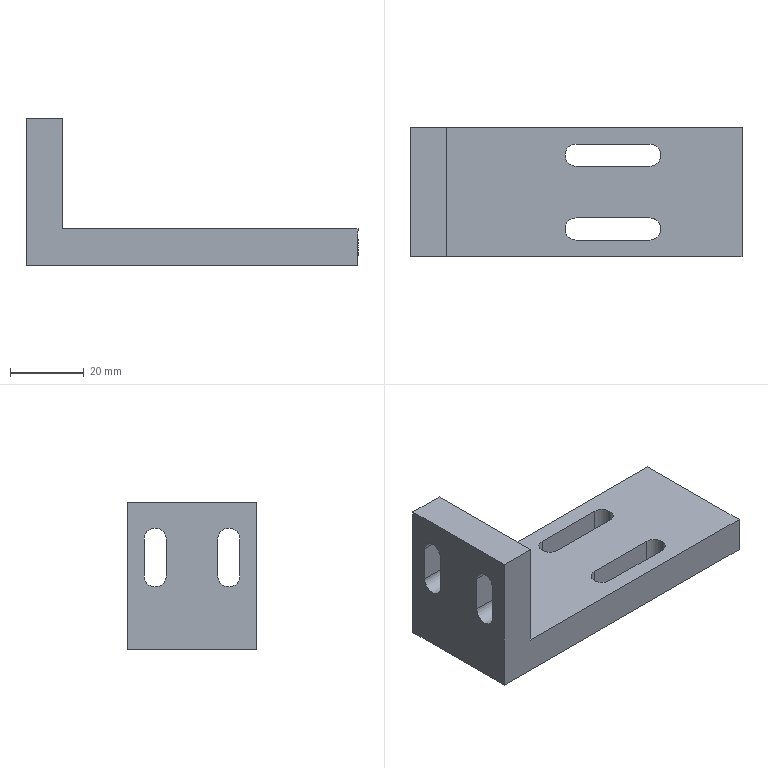Component | SolidWorks | ElectricalBoxAssembly2-1_AngleSensorComponentAssembly3-1_AdjustmentSeat-1 | 1 solid | 34 faces | box 90 x 35 x 40 mm | volume 36914 mm3 | plane 16 | cylinder 14 | cone 4 | commonest cylinder face diameters 6 x10 4.2 x4
build123d program:
from build123d import *

# Parameters (mm, degrees)
BOSS_EXTRUDE1_DEPTH   = 17.5
CUT_EXTRUDE1_DEPTH    = 92.139
CUT_EXTRUDE2_DEPTH    = 97.469
M5_TAPPED_HOLE1_D     = 4.2
M5_TAPPED_HOLE1_DEPTH = 12.4
M5_TAPPED_HOLE1_TIP   = 1.262


with BuildPart() as part:
    # Sketch1 → Boss-Extrude1 (new, symmetric)
    with BuildSketch(Plane.XY):
        Polygon((0, 0), (0, 90), (10, 90), (10, 10), (40, 10), (40, 0), align=None)
    extrude(amount=BOSS_EXTRUDE1_DEPTH, both=True)

    # Sketch2 → Cut-Extrude1 (cut, through all)
    with BuildSketch(Plane(origin=(0, 10, 0), x_dir=(1, 0, 0), z_dir=(0, 1, 0))):
        with BuildLine():
            Line((20, 13), (30, 13))
            ThreePointArc((30, 13), (33, 10), (30, 7))
            Line((30, 7), (20, 7))
            ThreePointArc((20, 7), (17, 10), (20, 13))
        make_face()
        with BuildLine():
            Line((20, -7), (30, -7))
            ThreePointArc((30, -7), (33, -10), (30, -13))
            Line((30, -13), (20, -13))
            ThreePointArc((20, -13), (17, -10), (20, -7))
        make_face()
    extrude(amount=-CUT_EXTRUDE1_DEPTH, mode=Mode.SUBTRACT)

    # Sketch3 → Cut-Extrude2 (cut, through all)
    with BuildSketch(Plane(origin=(10, 0, 0), x_dir=(0, 0, -1), z_dir=(1, 0, 0))):
        with BuildLine():
            Line((-7, 65), (-7, 45))
            ThreePointArc((-7, 45), (-10, 42), (-13, 45))
            Line((-13, 45), (-13, 65))
            ThreePointArc((-13, 65), (-10, 68), (-7, 65))
        make_face()
        with BuildLine():
            Line((13, 65), (13, 45))
            ThreePointArc((13, 45), (10, 42), (7, 45))
            Line((7, 45), (7, 65))
            ThreePointArc((7, 65), (10, 68), (13, 65))
        make_face()
    extrude(amount=-CUT_EXTRUDE2_DEPTH, mode=Mode.SUBTRACT)

    # M5 Tapped Hole1
    with Locations(Plane(origin=(0, 90, 0), x_dir=(1, 0, 0), z_dir=(0, 1, 0))):
        with Locations((5, 10), (5, -10)):
            Hole(M5_TAPPED_HOLE1_D / 2, depth=M5_TAPPED_HOLE1_DEPTH)
            with Locations((0, 0, -(M5_TAPPED_HOLE1_DEPTH + M5_TAPPED_HOLE1_TIP / 2))):  # 118° drill point
                Cone(0, M5_TAPPED_HOLE1_D / 2, M5_TAPPED_HOLE1_TIP, mode=Mode.SUBTRACT)


solid = part.part

# Placed as in the assembly
solid = solid.moved(Location((769.115, 214.666, 1766.399), (-90, 0, -90)))
STEP:
#1=COLOUR_RGB('',0.7922,0.8196,0.9333);
#2=FILL_AREA_STYLE_COLOUR('',#1);
#3=FILL_AREA_STYLE('',(#2));
#4=SURFACE_STYLE_FILL_AREA(#3);
#5=SURFACE_SIDE_STYLE('',(#4));
#6=SURFACE_STYLE_USAGE(.BOTH.,#5);
#7=PRESENTATION_STYLE_ASSIGNMENT((#6));
#8=CARTESIAN_POINT('',(33.335,7.975,69.74));
#9=VERTEX_POINT('',#8);
#10=CARTESIAN_POINT('',(33.335,8.14,69.74));
#11=VERTEX_POINT('',#10);
#12=CARTESIAN_POINT('',(33.335,8.058,69.74));
#13=DIRECTION('',(1.,0.,-0.));
#14=DIRECTION('',(0.,1.,0.));
#15=AXIS2_PLACEMENT_3D('',#12,#13,#14);
#16=CIRCLE('',#15,0.08268);
#17=EDGE_CURVE('',#9,#11,#16,.T.);
#18=ORIENTED_EDGE('',*,*,#17,.F.);
#19=CARTESIAN_POINT('',(33.823,7.975,69.74));
#20=VERTEX_POINT('',#19);
#21=CARTESIAN_POINT('',(33.823,7.975,69.74));
#22=DIRECTION('',(1.,0.,-0.));
#23=VECTOR('',#22,39.37);
#24=LINE('',#21,#23);
#25=EDGE_CURVE('',#9,#20,#24,.T.);
#26=ORIENTED_EDGE('',*,*,#25,.T.);
#27=CARTESIAN_POINT('',(33.823,8.14,69.74));
#28=VERTEX_POINT('',#27);
#29=CARTESIAN_POINT('',(33.823,8.058,69.74));
#30=DIRECTION('',(1.,0.,-0.));
#31=DIRECTION('',(0.,1.,0.));
#32=AXIS2_PLACEMENT_3D('',#29,#30,#31);
#33=CIRCLE('',#32,0.08268);
#34=EDGE_CURVE('',#20,#28,#33,.T.);
#35=ORIENTED_EDGE('',*,*,#34,.T.);
#36=CARTESIAN_POINT('',(33.823,8.14,69.74));
#37=DIRECTION('',(1.,0.,-0.));
#38=VECTOR('',#37,39.37);
#39=LINE('',#36,#38);
#40=EDGE_CURVE('',#11,#28,#39,.T.);
#41=ORIENTED_EDGE('',*,*,#40,.F.);
#42=EDGE_LOOP('',(#18,#26,#35,#41));
#43=FACE_OUTER_BOUND('',#42,.T.);
#44=CARTESIAN_POINT('',(33.823,8.058,69.74));
#45=DIRECTION('',(1.,0.,-0.));
#46=DIRECTION('',(0.,1.,0.));
#47=AXIS2_PLACEMENT_3D('',#44,#45,#46);
#48=CYLINDRICAL_SURFACE('',#47,0.08268);
#49=ADVANCED_FACE('',(#43),#48,.F.);
#50=CARTESIAN_POINT('',(33.286,8.058,69.74));
#51=VERTEX_POINT('',#50);
#52=CARTESIAN_POINT('',(33.335,8.14,69.74));
#53=DIRECTION('',(0.515,0.8572,-0.));
#54=VECTOR('',#53,39.37);
#55=LINE('',#52,#54);
#56=EDGE_CURVE('',#51,#11,#55,.T.);
#57=ORIENTED_EDGE('',*,*,#56,.F.);
#58=CARTESIAN_POINT('',(33.335,7.975,69.74));
#59=DIRECTION('',(0.515,-0.8572,-0.));
#60=VECTOR('',#59,39.37);
#61=LINE('',#58,#60);
#62=EDGE_CURVE('',#51,#9,#61,.T.);
#63=ORIENTED_EDGE('',*,*,#62,.T.);
#64=ORIENTED_EDGE('',*,*,#17,.T.);
#65=EDGE_LOOP('',(#57,#63,#64));
#66=FACE_OUTER_BOUND('',#65,.T.);
#67=CARTESIAN_POINT('',(33.335,8.058,69.74));
#68=DIRECTION('',(1.,0.,-0.));
#69=DIRECTION('',(0.,1.,0.));
#70=AXIS2_PLACEMENT_3D('',#67,#68,#69);
#71=CONICAL_SURFACE('',#70,0.08268,1.03);
#72=ADVANCED_FACE('',(#66),#71,.F.);
#73=CARTESIAN_POINT('',(33.335,8.762,69.74));
#74=VERTEX_POINT('',#73);
#75=CARTESIAN_POINT('',(33.335,8.928,69.74));
#76=VERTEX_POINT('',#75);
#77=CARTESIAN_POINT('',(33.335,8.845,69.74));
#78=DIRECTION('',(1.,0.,-0.));
#79=DIRECTION('',(0.,1.,0.));
#80=AXIS2_PLACEMENT_3D('',#77,#78,#79);
#81=CIRCLE('',#80,0.08268);
#82=EDGE_CURVE('',#74,#76,#81,.T.);
#83=ORIENTED_EDGE('',*,*,#82,.F.);
#84=CARTESIAN_POINT('',(33.823,8.762,69.74));
#85=VERTEX_POINT('',#84);
#86=CARTESIAN_POINT('',(33.823,8.762,69.74));
#87=DIRECTION('',(1.,0.,-0.));
#88=VECTOR('',#87,39.37);
#89=LINE('',#86,#88);
#90=EDGE_CURVE('',#74,#85,#89,.T.);
#91=ORIENTED_EDGE('',*,*,#90,.T.);
#92=CARTESIAN_POINT('',(33.823,8.928,69.74));
#93=VERTEX_POINT('',#92);
#94=CARTESIAN_POINT('',(33.823,8.845,69.74));
#95=DIRECTION('',(1.,0.,-0.));
#96=DIRECTION('',(0.,1.,0.));
#97=AXIS2_PLACEMENT_3D('',#94,#95,#96);
#98=CIRCLE('',#97,0.08268);
#99=EDGE_CURVE('',#85,#93,#98,.T.);
#100=ORIENTED_EDGE('',*,*,#99,.T.);
#101=CARTESIAN_POINT('',(33.823,8.928,69.74));
#102=DIRECTION('',(1.,0.,-0.));
#103=VECTOR('',#102,39.37);
#104=LINE('',#101,#103);
#105=EDGE_CURVE('',#76,#93,#104,.T.);
#106=ORIENTED_EDGE('',*,*,#105,.F.);
#107=EDGE_LOOP('',(#83,#91,#100,#106));
#108=FACE_OUTER_BOUND('',#107,.T.);
#109=CARTESIAN_POINT('',(33.823,8.845,69.74));
#110=DIRECTION('',(1.,0.,-0.));
#111=DIRECTION('',(0.,1.,0.));
#112=AXIS2_PLACEMENT_3D('',#109,#110,#111);
#113=CYLINDRICAL_SURFACE('',#112,0.08268);
#114=ADVANCED_FACE('',(#108),#113,.F.);
#115=CARTESIAN_POINT('',(33.286,8.845,69.74));
#116=VERTEX_POINT('',#115);
#117=CARTESIAN_POINT('',(33.335,8.928,69.74));
#118=DIRECTION('',(0.515,0.8572,-0.));
#119=VECTOR('',#118,39.37);
#120=LINE('',#117,#119);
#121=EDGE_CURVE('',#116,#76,#120,.T.);
#122=ORIENTED_EDGE('',*,*,#121,.F.);
#123=CARTESIAN_POINT('',(33.335,8.762,69.74));
#124=DIRECTION('',(0.515,-0.8572,-0.));
#125=VECTOR('',#124,39.37);
#126=LINE('',#123,#125);
#127=EDGE_CURVE('',#116,#74,#126,.T.);
#128=ORIENTED_EDGE('',*,*,#127,.T.);
#129=ORIENTED_EDGE('',*,*,#82,.T.);
#130=EDGE_LOOP('',(#122,#128,#129));
#131=FACE_OUTER_BOUND('',#130,.T.);
#132=CARTESIAN_POINT('',(33.335,8.845,69.74));
#133=DIRECTION('',(1.,0.,-0.));
#134=DIRECTION('',(0.,1.,0.));
#135=AXIS2_PLACEMENT_3D('',#132,#133,#134);
#136=CONICAL_SURFACE('',#135,0.08268,1.03);
#137=ADVANCED_FACE('',(#131),#136,.F.);
#138=CARTESIAN_POINT('',(32.957,8.058,69.543));
#139=VERTEX_POINT('',#138);
#140=CARTESIAN_POINT('',(32.839,8.176,69.543));
#141=VERTEX_POINT('',#140);
#142=CARTESIAN_POINT('',(32.839,8.058,69.543));
#143=DIRECTION('',(0.,0.,1.));
#144=DIRECTION('',(1.,0.,0.));
#145=AXIS2_PLACEMENT_3D('',#142,#143,#144);
#146=CIRCLE('',#145,0.1181);
#147=EDGE_CURVE('',#139,#141,#146,.T.);
#148=ORIENTED_EDGE('',*,*,#147,.F.);
#149=CARTESIAN_POINT('',(32.957,8.058,69.937));
#150=VERTEX_POINT('',#149);
#151=CARTESIAN_POINT('',(32.957,8.058,69.543));
#152=DIRECTION('',(0.,0.,1.));
#153=VECTOR('',#152,39.37);
#154=LINE('',#151,#153);
#155=EDGE_CURVE('',#139,#150,#154,.T.);
#156=ORIENTED_EDGE('',*,*,#155,.T.);
#157=CARTESIAN_POINT('',(32.839,8.176,69.937));
#158=VERTEX_POINT('',#157);
#159=CARTESIAN_POINT('',(32.839,8.058,69.937));
#160=DIRECTION('',(0.,0.,1.));
#161=DIRECTION('',(1.,0.,0.));
#162=AXIS2_PLACEMENT_3D('',#159,#160,#161);
#163=CIRCLE('',#162,0.1181);
#164=EDGE_CURVE('',#150,#158,#163,.T.);
#165=ORIENTED_EDGE('',*,*,#164,.T.);
#166=CARTESIAN_POINT('',(32.839,8.176,69.543));
#167=DIRECTION('',(0.,0.,1.));
#168=VECTOR('',#167,39.37);
#169=LINE('',#166,#168);
#170=EDGE_CURVE('',#141,#158,#169,.T.);
#171=ORIENTED_EDGE('',*,*,#170,.F.);
#172=EDGE_LOOP('',(#148,#156,#165,#171));
#173=FACE_OUTER_BOUND('',#172,.T.);
#174=CARTESIAN_POINT('',(32.839,8.058,69.543));
#175=DIRECTION('',(0.,0.,1.));
#176=DIRECTION('',(1.,0.,0.));
#177=AXIS2_PLACEMENT_3D('',#174,#175,#176);
#178=CYLINDRICAL_SURFACE('',#177,0.1181);
#179=ADVANCED_FACE('',(#173),#178,.F.);
#180=CARTESIAN_POINT('',(32.957,8.845,69.543));
#181=VERTEX_POINT('',#180);
#182=CARTESIAN_POINT('',(32.839,8.963,69.543));
#183=VERTEX_POINT('',#182);
#184=CARTESIAN_POINT('',(32.839,8.845,69.543));
#185=DIRECTION('',(0.,0.,1.));
#186=DIRECTION('',(1.,0.,0.));
#187=AXIS2_PLACEMENT_3D('',#184,#185,#186);
#188=CIRCLE('',#187,0.1181);
#189=EDGE_CURVE('',#181,#183,#188,.T.);
#190=ORIENTED_EDGE('',*,*,#189,.F.);
#191=CARTESIAN_POINT('',(32.957,8.845,69.937));
#192=VERTEX_POINT('',#191);
#193=CARTESIAN_POINT('',(32.957,8.845,69.543));
#194=DIRECTION('',(0.,0.,1.));
#195=VECTOR('',#194,39.37);
#196=LINE('',#193,#195);
#197=EDGE_CURVE('',#181,#192,#196,.T.);
#198=ORIENTED_EDGE('',*,*,#197,.T.);
#199=CARTESIAN_POINT('',(32.839,8.963,69.937));
#200=VERTEX_POINT('',#199);
#201=CARTESIAN_POINT('',(32.839,8.845,69.937));
#202=DIRECTION('',(0.,0.,1.));
#203=DIRECTION('',(1.,0.,0.));
#204=AXIS2_PLACEMENT_3D('',#201,#202,#203);
#205=CIRCLE('',#204,0.1181);
#206=EDGE_CURVE('',#192,#200,#205,.T.);
#207=ORIENTED_EDGE('',*,*,#206,.T.);
#208=CARTESIAN_POINT('',(32.839,8.963,69.543));
#209=DIRECTION('',(0.,0.,1.));
#210=VECTOR('',#209,39.37);
#211=LINE('',#208,#210);
#212=EDGE_CURVE('',#183,#200,#211,.T.);
#213=ORIENTED_EDGE('',*,*,#212,.F.);
#214=EDGE_LOOP('',(#190,#198,#207,#213));
#215=FACE_OUTER_BOUND('',#214,.T.);
#216=CARTESIAN_POINT('',(32.839,8.845,69.543));
#217=DIRECTION('',(0.,0.,1.));
#218=DIRECTION('',(1.,0.,0.));
#219=AXIS2_PLACEMENT_3D('',#216,#217,#218);
#220=CYLINDRICAL_SURFACE('',#219,0.1181);
#221=ADVANCED_FACE('',(#215),#220,.F.);
#222=CARTESIAN_POINT('',(30.28,8.727,70.724));
#223=VERTEX_POINT('',#222);
#224=CARTESIAN_POINT('',(30.28,8.727,70.331));
#225=VERTEX_POINT('',#224);
#226=CARTESIAN_POINT('',(30.28,8.727,70.331));
#227=DIRECTION('',(-0.,-0.,-1.));
#228=VECTOR('',#227,39.37);
#229=LINE('',#226,#228);
#230=EDGE_CURVE('',#223,#225,#229,.T.);
#231=ORIENTED_EDGE('',*,*,#230,.T.);
#232=CARTESIAN_POINT('',(30.28,8.963,70.331));
#233=VERTEX_POINT('',#232);
#234=CARTESIAN_POINT('',(30.28,8.845,70.331));
#235=DIRECTION('',(1.,0.,-0.));
#236=DIRECTION('',(0.,1.,0.));
#237=AXIS2_PLACEMENT_3D('',#234,#235,#236);
#238=CIRCLE('',#237,0.1181);
#239=EDGE_CURVE('',#225,#233,#238,.T.);
#240=ORIENTED_EDGE('',*,*,#239,.T.);
#241=CARTESIAN_POINT('',(30.28,8.963,70.724));
#242=VERTEX_POINT('',#241);
#243=CARTESIAN_POINT('',(30.28,8.963,70.331));
#244=DIRECTION('',(0.,0.,1.));
#245=VECTOR('',#244,39.37);
#246=LINE('',#243,#245);
#247=EDGE_CURVE('',#233,#242,#246,.T.);
#248=ORIENTED_EDGE('',*,*,#247,.T.);
#249=CARTESIAN_POINT('',(30.28,8.845,70.724));
#250=DIRECTION('',(1.,0.,-0.));
#251=DIRECTION('',(0.,1.,0.));
#252=AXIS2_PLACEMENT_3D('',#249,#250,#251);
#253=CIRCLE('',#252,0.1181);
#254=EDGE_CURVE('',#242,#223,#253,.T.);
#255=ORIENTED_EDGE('',*,*,#254,.T.);
#256=EDGE_LOOP('',(#231,#240,#248,#255));
#257=FACE_BOUND('',#256,.T.);
#258=CARTESIAN_POINT('',(30.28,7.94,70.724));
#259=VERTEX_POINT('',#258);
#260=CARTESIAN_POINT('',(30.28,7.94,70.331));
#261=VERTEX_POINT('',#260);
#262=CARTESIAN_POINT('',(30.28,7.94,70.331));
#263=DIRECTION('',(-0.,-0.,-1.));
#264=VECTOR('',#263,39.37);
#265=LINE('',#262,#264);
#266=EDGE_CURVE('',#259,#261,#265,.T.);
#267=ORIENTED_EDGE('',*,*,#266,.T.);
#268=CARTESIAN_POINT('',(30.28,8.176,70.331));
#269=VERTEX_POINT('',#268);
#270=CARTESIAN_POINT('',(30.28,8.058,70.331));
#271=DIRECTION('',(1.,0.,-0.));
#272=DIRECTION('',(0.,1.,0.));
#273=AXIS2_PLACEMENT_3D('',#270,#271,#272);
#274=CIRCLE('',#273,0.1181);
#275=EDGE_CURVE('',#261,#269,#274,.T.);
#276=ORIENTED_EDGE('',*,*,#275,.T.);
#277=CARTESIAN_POINT('',(30.28,8.176,70.724));
#278=VERTEX_POINT('',#277);
#279=CARTESIAN_POINT('',(30.28,8.176,70.331));
#280=DIRECTION('',(0.,0.,1.));
#281=VECTOR('',#280,39.37);
#282=LINE('',#279,#281);
#283=EDGE_CURVE('',#269,#278,#282,.T.);
#284=ORIENTED_EDGE('',*,*,#283,.T.);
#285=CARTESIAN_POINT('',(30.28,8.058,70.724));
#286=DIRECTION('',(1.,0.,-0.));
#287=DIRECTION('',(0.,1.,0.));
#288=AXIS2_PLACEMENT_3D('',#285,#286,#287);
#289=CIRCLE('',#288,0.1181);
#290=EDGE_CURVE('',#278,#259,#289,.T.);
#291=ORIENTED_EDGE('',*,*,#290,.T.);
#292=EDGE_LOOP('',(#267,#276,#284,#291));
#293=FACE_BOUND('',#292,.T.);
#294=CARTESIAN_POINT('',(30.28,7.762,69.543));
#295=VERTEX_POINT('',#294);
#296=CARTESIAN_POINT('',(30.28,7.762,71.118));
#297=VERTEX_POINT('',#296);
#298=CARTESIAN_POINT('',(30.28,7.762,71.118));
#299=DIRECTION('',(0.,0.,1.));
#300=VECTOR('',#299,39.37);
#301=LINE('',#298,#300);
#302=EDGE_CURVE('',#295,#297,#301,.T.);
#303=ORIENTED_EDGE('',*,*,#302,.T.);
#304=CARTESIAN_POINT('',(30.28,9.14,71.118));
#305=VERTEX_POINT('',#304);
#306=CARTESIAN_POINT('',(30.28,9.14,71.118));
#307=DIRECTION('',(0.,-1.,0.));
#308=VECTOR('',#307,39.37);
#309=LINE('',#306,#308);
#310=EDGE_CURVE('',#305,#297,#309,.T.);
#311=ORIENTED_EDGE('',*,*,#310,.F.);
#312=CARTESIAN_POINT('',(30.28,9.14,69.543));
#313=VERTEX_POINT('',#312);
#314=CARTESIAN_POINT('',(30.28,9.14,71.118));
#315=DIRECTION('',(0.,0.,1.));
#316=VECTOR('',#315,39.37);
#317=LINE('',#314,#316);
#318=EDGE_CURVE('',#313,#305,#317,.T.);
#319=ORIENTED_EDGE('',*,*,#318,.F.);
#320=CARTESIAN_POINT('',(30.28,9.14,69.543));
#321=DIRECTION('',(0.,-1.,0.));
#322=VECTOR('',#321,39.37);
#323=LINE('',#320,#322);
#324=EDGE_CURVE('',#313,#295,#323,.T.);
#325=ORIENTED_EDGE('',*,*,#324,.T.);
#326=EDGE_LOOP('',(#303,#311,#319,#325));
#327=FACE_OUTER_BOUND('',#326,.T.);
#328=CARTESIAN_POINT('',(30.28,9.14,71.118));
#329=DIRECTION('',(1.,0.,-0.));
#330=DIRECTION('',(-0.,-0.,-1.));
#331=AXIS2_PLACEMENT_3D('',#328,#329,#330);
#332=PLANE('',#331);
#333=ADVANCED_FACE('',(#257,#293,#327),#332,.F.);
#334=CARTESIAN_POINT('',(30.674,7.762,71.118));
#335=VERTEX_POINT('',#334);
#336=CARTESIAN_POINT('',(30.674,7.762,71.118));
#337=DIRECTION('',(1.,0.,-0.));
#338=VECTOR('',#337,39.37);
#339=LINE('',#336,#338);
#340=EDGE_CURVE('',#297,#335,#339,.T.);
#341=ORIENTED_EDGE('',*,*,#340,.T.);
#342=CARTESIAN_POINT('',(30.674,9.14,71.118));
#343=VERTEX_POINT('',#342);
#344=CARTESIAN_POINT('',(30.674,9.14,71.118));
#345=DIRECTION('',(0.,-1.,0.));
#346=VECTOR('',#345,39.37);
#347=LINE('',#344,#346);
#348=EDGE_CURVE('',#343,#335,#347,.T.);
#349=ORIENTED_EDGE('',*,*,#348,.F.);
#350=CARTESIAN_POINT('',(30.674,9.14,71.118));
#351=DIRECTION('',(1.,0.,-0.));
#352=VECTOR('',#351,39.37);
#353=LINE('',#350,#352);
#354=EDGE_CURVE('',#305,#343,#353,.T.);
#355=ORIENTED_EDGE('',*,*,#354,.F.);
#356=ORIENTED_EDGE('',*,*,#310,.T.);
#357=EDGE_LOOP('',(#341,#349,#355,#356));
#358=FACE_OUTER_BOUND('',#357,.T.);
#359=CARTESIAN_POINT('',(30.674,9.14,71.118));
#360=DIRECTION('',(-0.,-0.,-1.));
#361=DIRECTION('',(-0.,1.,-0.));
#362=AXIS2_PLACEMENT_3D('',#359,#360,#361);
#363=PLANE('',#362);
#364=ADVANCED_FACE('',(#358),#363,.F.);
#365=CARTESIAN_POINT('',(30.674,8.963,70.331));
#366=VERTEX_POINT('',#365);
#367=CARTESIAN_POINT('',(30.674,8.963,70.724));
#368=VERTEX_POINT('',#367);
#369=CARTESIAN_POINT('',(30.674,8.963,70.331));
#370=DIRECTION('',(0.,0.,1.));
#371=VECTOR('',#370,39.37);
#372=LINE('',#369,#371);
#373=EDGE_CURVE('',#366,#368,#372,.T.);
#374=ORIENTED_EDGE('',*,*,#373,.F.);
#375=CARTESIAN_POINT('',(30.674,8.727,70.331));
#376=VERTEX_POINT('',#375);
#377=CARTESIAN_POINT('',(30.674,8.845,70.331));
#378=DIRECTION('',(1.,0.,-0.));
#379=DIRECTION('',(0.,1.,0.));
#380=AXIS2_PLACEMENT_3D('',#377,#378,#379);
#381=CIRCLE('',#380,0.1181);
#382=EDGE_CURVE('',#376,#366,#381,.T.);
#383=ORIENTED_EDGE('',*,*,#382,.F.);
#384=CARTESIAN_POINT('',(30.674,8.727,70.724));
#385=VERTEX_POINT('',#384);
#386=CARTESIAN_POINT('',(30.674,8.727,70.331));
#387=DIRECTION('',(-0.,-0.,-1.));
#388=VECTOR('',#387,39.37);
#389=LINE('',#386,#388);
#390=EDGE_CURVE('',#385,#376,#389,.T.);
#391=ORIENTED_EDGE('',*,*,#390,.F.);
#392=CARTESIAN_POINT('',(30.674,8.845,70.724));
#393=DIRECTION('',(1.,0.,-0.));
#394=DIRECTION('',(0.,1.,0.));
#395=AXIS2_PLACEMENT_3D('',#392,#393,#394);
#396=CIRCLE('',#395,0.1181);
#397=EDGE_CURVE('',#368,#385,#396,.T.);
#398=ORIENTED_EDGE('',*,*,#397,.F.);
#399=EDGE_LOOP('',(#374,#383,#391,#398));
#400=FACE_BOUND('',#399,.T.);
#401=CARTESIAN_POINT('',(30.674,8.176,70.331));
#402=VERTEX_POINT('',#401);
#403=CARTESIAN_POINT('',(30.674,8.176,70.724));
#404=VERTEX_POINT('',#403);
#405=CARTESIAN_POINT('',(30.674,8.176,70.331));
#406=DIRECTION('',(0.,0.,1.));
#407=VECTOR('',#406,39.37);
#408=LINE('',#405,#407);
#409=EDGE_CURVE('',#402,#404,#408,.T.);
#410=ORIENTED_EDGE('',*,*,#409,.F.);
#411=CARTESIAN_POINT('',(30.674,7.94,70.331));
#412=VERTEX_POINT('',#411);
#413=CARTESIAN_POINT('',(30.674,8.058,70.331));
#414=DIRECTION('',(1.,0.,-0.));
#415=DIRECTION('',(0.,1.,0.));
#416=AXIS2_PLACEMENT_3D('',#413,#414,#415);
#417=CIRCLE('',#416,0.1181);
#418=EDGE_CURVE('',#412,#402,#417,.T.);
#419=ORIENTED_EDGE('',*,*,#418,.F.);
#420=CARTESIAN_POINT('',(30.674,7.94,70.724));
#421=VERTEX_POINT('',#420);
#422=CARTESIAN_POINT('',(30.674,7.94,70.331));
#423=DIRECTION('',(-0.,-0.,-1.));
#424=VECTOR('',#423,39.37);
#425=LINE('',#422,#424);
#426=EDGE_CURVE('',#421,#412,#425,.T.);
#427=ORIENTED_EDGE('',*,*,#426,.F.);
#428=CARTESIAN_POINT('',(30.674,8.058,70.724));
#429=DIRECTION('',(1.,0.,-0.));
#430=DIRECTION('',(0.,1.,0.));
#431=AXIS2_PLACEMENT_3D('',#428,#429,#430);
#432=CIRCLE('',#431,0.1181);
#433=EDGE_CURVE('',#404,#421,#432,.T.);
#434=ORIENTED_EDGE('',*,*,#433,.F.);
#435=EDGE_LOOP('',(#410,#419,#427,#434));
#436=FACE_BOUND('',#435,.T.);
#437=CARTESIAN_POINT('',(30.674,7.762,69.937));
#438=VERTEX_POINT('',#437);
#439=CARTESIAN_POINT('',(30.674,7.762,69.937));
#440=DIRECTION('',(-0.,-0.,-1.));
#441=VECTOR('',#440,39.37);
#442=LINE('',#439,#441);
#443=EDGE_CURVE('',#335,#438,#442,.T.);
#444=ORIENTED_EDGE('',*,*,#443,.T.);
#445=CARTESIAN_POINT('',(30.674,9.14,69.937));
#446=VERTEX_POINT('',#445);
#447=CARTESIAN_POINT('',(30.674,9.14,69.937));
#448=DIRECTION('',(0.,-1.,0.));
#449=VECTOR('',#448,39.37);
#450=LINE('',#447,#449);
#451=EDGE_CURVE('',#446,#438,#450,.T.);
#452=ORIENTED_EDGE('',*,*,#451,.F.);
#453=CARTESIAN_POINT('',(30.674,9.14,69.937));
#454=DIRECTION('',(-0.,-0.,-1.));
#455=VECTOR('',#454,39.37);
#456=LINE('',#453,#455);
#457=EDGE_CURVE('',#343,#446,#456,.T.);
#458=ORIENTED_EDGE('',*,*,#457,.F.);
#459=ORIENTED_EDGE('',*,*,#348,.T.);
#460=EDGE_LOOP('',(#444,#452,#458,#459));
#461=FACE_OUTER_BOUND('',#460,.T.);
#462=CARTESIAN_POINT('',(30.674,9.14,69.937));
#463=DIRECTION('',(-1.,0.,0.));
#464=DIRECTION('',(0.,-1.,0.));
#465=AXIS2_PLACEMENT_3D('',#462,#463,#464);
#466=PLANE('',#465);
#467=ADVANCED_FACE('',(#400,#436,#461),#466,.F.);
#468=CARTESIAN_POINT('',(32.052,8.176,69.937));
#469=VERTEX_POINT('',#468);
#470=CARTESIAN_POINT('',(32.839,8.176,69.937));
#471=DIRECTION('',(-1.,-0.,0.));
#472=VECTOR('',#471,39.37);
#473=LINE('',#470,#472);
#474=EDGE_CURVE('',#158,#469,#473,.T.);
#475=ORIENTED_EDGE('',*,*,#474,.F.);
#476=ORIENTED_EDGE('',*,*,#164,.F.);
#477=CARTESIAN_POINT('',(32.839,7.94,69.937));
#478=VERTEX_POINT('',#477);
#479=CARTESIAN_POINT('',(32.839,8.058,69.937));
#480=DIRECTION('',(0.,0.,1.));
#481=DIRECTION('',(1.,0.,0.));
#482=AXIS2_PLACEMENT_3D('',#479,#480,#481);
#483=CIRCLE('',#482,0.1181);
#484=EDGE_CURVE('',#478,#150,#483,.T.);
#485=ORIENTED_EDGE('',*,*,#484,.F.);
#486=CARTESIAN_POINT('',(32.052,7.94,69.937));
#487=VERTEX_POINT('',#486);
#488=CARTESIAN_POINT('',(32.839,7.94,69.937));
#489=DIRECTION('',(1.,0.,-0.));
#490=VECTOR('',#489,39.37);
#491=LINE('',#488,#490);
#492=EDGE_CURVE('',#487,#478,#491,.T.);
#493=ORIENTED_EDGE('',*,*,#492,.F.);
#494=CARTESIAN_POINT('',(32.052,8.058,69.937));
#495=DIRECTION('',(0.,0.,1.));
#496=DIRECTION('',(1.,0.,0.));
#497=AXIS2_PLACEMENT_3D('',#494,#495,#496);
#498=CIRCLE('',#497,0.1181);
#499=EDGE_CURVE('',#469,#487,#498,.T.);
#500=ORIENTED_EDGE('',*,*,#499,.F.);
#501=EDGE_LOOP('',(#475,#476,#485,#493,#500));
#502=FACE_BOUND('',#501,.T.);
#503=CARTESIAN_POINT('',(32.052,8.963,69.937));
#504=VERTEX_POINT('',#503);
#505=CARTESIAN_POINT('',(32.839,8.963,69.937));
#506=DIRECTION('',(-1.,-0.,0.));
#507=VECTOR('',#506,39.37);
#508=LINE('',#505,#507);
#509=EDGE_CURVE('',#200,#504,#508,.T.);
#510=ORIENTED_EDGE('',*,*,#509,.F.);
#511=ORIENTED_EDGE('',*,*,#206,.F.);
#512=CARTESIAN_POINT('',(32.839,8.727,69.937));
#513=VERTEX_POINT('',#512);
#514=CARTESIAN_POINT('',(32.839,8.845,69.937));
#515=DIRECTION('',(0.,0.,1.));
#516=DIRECTION('',(1.,0.,0.));
#517=AXIS2_PLACEMENT_3D('',#514,#515,#516);
#518=CIRCLE('',#517,0.1181);
#519=EDGE_CURVE('',#513,#192,#518,.T.);
#520=ORIENTED_EDGE('',*,*,#519,.F.);
#521=CARTESIAN_POINT('',(32.052,8.727,69.937));
#522=VERTEX_POINT('',#521);
#523=CARTESIAN_POINT('',(32.839,8.727,69.937));
#524=DIRECTION('',(1.,0.,-0.));
#525=VECTOR('',#524,39.37);
#526=LINE('',#523,#525);
#527=EDGE_CURVE('',#522,#513,#526,.T.);
#528=ORIENTED_EDGE('',*,*,#527,.F.);
#529=CARTESIAN_POINT('',(32.052,8.845,69.937));
#530=DIRECTION('',(0.,0.,1.));
#531=DIRECTION('',(1.,0.,0.));
#532=AXIS2_PLACEMENT_3D('',#529,#530,#531);
#533=CIRCLE('',#532,0.1181);
#534=EDGE_CURVE('',#504,#522,#533,.T.);
#535=ORIENTED_EDGE('',*,*,#534,.F.);
#536=EDGE_LOOP('',(#510,#511,#520,#528,#535));
#537=FACE_BOUND('',#536,.T.);
#538=CARTESIAN_POINT('',(33.823,7.762,69.937));
#539=VERTEX_POINT('',#538);
#540=CARTESIAN_POINT('',(33.823,7.762,69.937));
#541=DIRECTION('',(1.,0.,-0.));
#542=VECTOR('',#541,39.37);
#543=LINE('',#540,#542);
#544=EDGE_CURVE('',#438,#539,#543,.T.);
#545=ORIENTED_EDGE('',*,*,#544,.T.);
#546=CARTESIAN_POINT('',(33.823,9.14,69.937));
#547=VERTEX_POINT('',#546);
#548=CARTESIAN_POINT('',(33.823,9.14,69.937));
#549=DIRECTION('',(0.,-1.,0.));
#550=VECTOR('',#549,39.37);
#551=LINE('',#548,#550);
#552=EDGE_CURVE('',#547,#539,#551,.T.);
#553=ORIENTED_EDGE('',*,*,#552,.F.);
#554=CARTESIAN_POINT('',(33.823,9.14,69.937));
#555=DIRECTION('',(1.,0.,-0.));
#556=VECTOR('',#555,39.37);
#557=LINE('',#554,#556);
#558=EDGE_CURVE('',#446,#547,#557,.T.);
#559=ORIENTED_EDGE('',*,*,#558,.F.);
#560=ORIENTED_EDGE('',*,*,#451,.T.);
#561=EDGE_LOOP('',(#545,#553,#559,#560));
#562=FACE_OUTER_BOUND('',#561,.T.);
#563=CARTESIAN_POINT('',(33.823,9.14,69.937));
#564=DIRECTION('',(-0.,-0.,-1.));
#565=DIRECTION('',(-1.,-0.,0.));
#566=AXIS2_PLACEMENT_3D('',#563,#564,#565);
#567=PLANE('',#566);
#568=ADVANCED_FACE('',(#502,#537,#562),#567,.F.);
#569=CARTESIAN_POINT('',(33.823,8.058,69.74));
#570=DIRECTION('',(1.,0.,-0.));
#571=DIRECTION('',(0.,1.,0.));
#572=AXIS2_PLACEMENT_3D('',#569,#570,#571);
#573=CIRCLE('',#572,0.08268);
#574=EDGE_CURVE('',#28,#20,#573,.T.);
#575=ORIENTED_EDGE('',*,*,#574,.F.);
#576=ORIENTED_EDGE('',*,*,#34,.F.);
#577=EDGE_LOOP('',(#575,#576));
#578=FACE_BOUND('',#577,.T.);
#579=CARTESIAN_POINT('',(33.823,8.845,69.74));
#580=DIRECTION('',(1.,0.,-0.));
#581=DIRECTION('',(0.,1.,0.));
#582=AXIS2_PLACEMENT_3D('',#579,#580,#581);
#583=CIRCLE('',#582,0.08268);
#584=EDGE_CURVE('',#93,#85,#583,.T.);
#585=ORIENTED_EDGE('',*,*,#584,.F.);
#586=ORIENTED_EDGE('',*,*,#99,.F.);
#587=EDGE_LOOP('',(#585,#586));
#588=FACE_BOUND('',#587,.T.);
#589=CARTESIAN_POINT('',(33.823,7.762,69.543));
#590=VERTEX_POINT('',#589);
#591=CARTESIAN_POINT('',(33.823,7.762,69.543));
#592=DIRECTION('',(-0.,-0.,-1.));
#593=VECTOR('',#592,39.37);
#594=LINE('',#591,#593);
#595=EDGE_CURVE('',#539,#590,#594,.T.);
#596=ORIENTED_EDGE('',*,*,#595,.T.);
#597=CARTESIAN_POINT('',(33.823,9.14,69.543));
#598=VERTEX_POINT('',#597);
#599=CARTESIAN_POINT('',(33.823,9.14,69.543));
#600=DIRECTION('',(0.,-1.,0.));
#601=VECTOR('',#600,39.37);
#602=LINE('',#599,#601);
#603=EDGE_CURVE('',#598,#590,#602,.T.);
#604=ORIENTED_EDGE('',*,*,#603,.F.);
#605=CARTESIAN_POINT('',(33.823,9.14,69.543));
#606=DIRECTION('',(-0.,-0.,-1.));
#607=VECTOR('',#606,39.37);
#608=LINE('',#605,#607);
#609=EDGE_CURVE('',#547,#598,#608,.T.);
#610=ORIENTED_EDGE('',*,*,#609,.F.);
#611=ORIENTED_EDGE('',*,*,#552,.T.);
#612=EDGE_LOOP('',(#596,#604,#610,#611));
#613=FACE_OUTER_BOUND('',#612,.T.);
#614=CARTESIAN_POINT('',(33.823,9.14,69.543));
#615=DIRECTION('',(-1.,0.,0.));
#616=DIRECTION('',(0.,-1.,0.));
#617=AXIS2_PLACEMENT_3D('',#614,#615,#616);
#618=PLANE('',#617);
#619=ADVANCED_FACE('',(#578,#588,#613),#618,.F.);
#620=CARTESIAN_POINT('',(32.052,7.94,69.543));
#621=VERTEX_POINT('',#620);
#622=CARTESIAN_POINT('',(32.839,7.94,69.543));
#623=VERTEX_POINT('',#622);
#624=CARTESIAN_POINT('',(32.839,7.94,69.543));
#625=DIRECTION('',(1.,0.,-0.));
#626=VECTOR('',#625,39.37);
#627=LINE('',#624,#626);
#628=EDGE_CURVE('',#621,#623,#627,.T.);
#629=ORIENTED_EDGE('',*,*,#628,.T.);
#630=CARTESIAN_POINT('',(32.839,8.058,69.543));
#631=DIRECTION('',(0.,0.,1.));
#632=DIRECTION('',(1.,0.,0.));
#633=AXIS2_PLACEMENT_3D('',#630,#631,#632);
#634=CIRCLE('',#633,0.1181);
#635=EDGE_CURVE('',#623,#139,#634,.T.);
#636=ORIENTED_EDGE('',*,*,#635,.T.);
#637=ORIENTED_EDGE('',*,*,#147,.T.);
#638=CARTESIAN_POINT('',(32.052,8.176,69.543));
#639=VERTEX_POINT('',#638);
#640=CARTESIAN_POINT('',(32.839,8.176,69.543));
#641=DIRECTION('',(-1.,-0.,0.));
#642=VECTOR('',#641,39.37);
#643=LINE('',#640,#642);
#644=EDGE_CURVE('',#141,#639,#643,.T.);
#645=ORIENTED_EDGE('',*,*,#644,.T.);
#646=CARTESIAN_POINT('',(32.052,8.058,69.543));
#647=DIRECTION('',(0.,0.,1.));
#648=DIRECTION('',(1.,0.,0.));
#649=AXIS2_PLACEMENT_3D('',#646,#647,#648);
#650=CIRCLE('',#649,0.1181);
#651=EDGE_CURVE('',#639,#621,#650,.T.);
#652=ORIENTED_EDGE('',*,*,#651,.T.);
#653=EDGE_LOOP('',(#629,#636,#637,#645,#652));
#654=FACE_BOUND('',#653,.T.);
#655=CARTESIAN_POINT('',(32.052,8.727,69.543));
#656=VERTEX_POINT('',#655);
#657=CARTESIAN_POINT('',(32.839,8.727,69.543));
#658=VERTEX_POINT('',#657);
#659=CARTESIAN_POINT('',(32.839,8.727,69.543));
#660=DIRECTION('',(1.,0.,-0.));
#661=VECTOR('',#660,39.37);
#662=LINE('',#659,#661);
#663=EDGE_CURVE('',#656,#658,#662,.T.);
#664=ORIENTED_EDGE('',*,*,#663,.T.);
#665=CARTESIAN_POINT('',(32.839,8.845,69.543));
#666=DIRECTION('',(0.,0.,1.));
#667=DIRECTION('',(1.,0.,0.));
#668=AXIS2_PLACEMENT_3D('',#665,#666,#667);
#669=CIRCLE('',#668,0.1181);
#670=EDGE_CURVE('',#658,#181,#669,.T.);
#671=ORIENTED_EDGE('',*,*,#670,.T.);
#672=ORIENTED_EDGE('',*,*,#189,.T.);
#673=CARTESIAN_POINT('',(32.052,8.963,69.543));
#674=VERTEX_POINT('',#673);
#675=CARTESIAN_POINT('',(32.839,8.963,69.543));
#676=DIRECTION('',(-1.,-0.,0.));
#677=VECTOR('',#676,39.37);
#678=LINE('',#675,#677);
#679=EDGE_CURVE('',#183,#674,#678,.T.);
#680=ORIENTED_EDGE('',*,*,#679,.T.);
#681=CARTESIAN_POINT('',(32.052,8.845,69.543));
#682=DIRECTION('',(0.,0.,1.));
#683=DIRECTION('',(1.,0.,0.));
#684=AXIS2_PLACEMENT_3D('',#681,#682,#683);
#685=CIRCLE('',#684,0.1181);
#686=EDGE_CURVE('',#674,#656,#685,.T.);
#687=ORIENTED_EDGE('',*,*,#686,.T.);
#688=EDGE_LOOP('',(#664,#671,#672,#680,#687));
#689=FACE_BOUND('',#688,.T.);
#690=CARTESIAN_POINT('',(30.28,7.762,69.543));
#691=DIRECTION('',(-1.,-0.,0.));
#692=VECTOR('',#691,39.37);
#693=LINE('',#690,#692);
#694=EDGE_CURVE('',#590,#295,#693,.T.);
#695=ORIENTED_EDGE('',*,*,#694,.T.);
#696=ORIENTED_EDGE('',*,*,#324,.F.);
#697=CARTESIAN_POINT('',(30.28,9.14,69.543));
#698=DIRECTION('',(-1.,-0.,0.));
#699=VECTOR('',#698,39.37);
#700=LINE('',#697,#699);
#701=EDGE_CURVE('',#598,#313,#700,.T.);
#702=ORIENTED_EDGE('',*,*,#701,.F.);
#703=ORIENTED_EDGE('',*,*,#603,.T.);
#704=EDGE_LOOP('',(#695,#696,#702,#703));
#705=FACE_OUTER_BOUND('',#704,.T.);
#706=CARTESIAN_POINT('',(30.28,9.14,69.543));
#707=DIRECTION('',(0.,0.,1.));
#708=DIRECTION('',(0.,-1.,0.));
#709=AXIS2_PLACEMENT_3D('',#706,#707,#708);
#710=PLANE('',#709);
#711=ADVANCED_FACE('',(#654,#689,#705),#710,.F.);
#712=ORIENTED_EDGE('',*,*,#318,.T.);
#713=ORIENTED_EDGE('',*,*,#354,.T.);
#714=ORIENTED_EDGE('',*,*,#457,.T.);
#715=ORIENTED_EDGE('',*,*,#558,.T.);
#716=ORIENTED_EDGE('',*,*,#609,.T.);
#717=ORIENTED_EDGE('',*,*,#701,.T.);
#718=EDGE_LOOP('',(#712,#713,#714,#715,#716,#717));
#719=FACE_OUTER_BOUND('',#718,.T.);
#720=CARTESIAN_POINT('',(30.28,9.14,69.543));
#721=DIRECTION('',(0.,-1.,0.));
#722=DIRECTION('',(-0.,-0.,-1.));
#723=AXIS2_PLACEMENT_3D('',#720,#721,#722);
#724=PLANE('',#723);
#725=ADVANCED_FACE('',(#719),#724,.F.);
#726=ORIENTED_EDGE('',*,*,#302,.F.);
#727=ORIENTED_EDGE('',*,*,#694,.F.);
#728=ORIENTED_EDGE('',*,*,#595,.F.);
#729=ORIENTED_EDGE('',*,*,#544,.F.);
#730=ORIENTED_EDGE('',*,*,#443,.F.);
#731=ORIENTED_EDGE('',*,*,#340,.F.);
#732=EDGE_LOOP('',(#726,#727,#728,#729,#730,#731));
#733=FACE_OUTER_BOUND('',#732,.T.);
#734=CARTESIAN_POINT('',(30.28,7.762,69.543));
#735=DIRECTION('',(0.,-1.,0.));
#736=DIRECTION('',(-0.,-0.,-1.));
#737=AXIS2_PLACEMENT_3D('',#734,#735,#736);
#738=PLANE('',#737);
#739=ADVANCED_FACE('',(#733),#738,.T.);
#740=ORIENTED_EDGE('',*,*,#418,.T.);
#741=CARTESIAN_POINT('',(30.28,8.176,70.331));
#742=DIRECTION('',(1.,0.,-0.));
#743=VECTOR('',#742,39.37);
#744=LINE('',#741,#743);
#745=EDGE_CURVE('',#269,#402,#744,.T.);
#746=ORIENTED_EDGE('',*,*,#745,.F.);
#747=ORIENTED_EDGE('',*,*,#275,.F.);
#748=CARTESIAN_POINT('',(30.28,7.94,70.331));
#749=DIRECTION('',(1.,0.,-0.));
#750=VECTOR('',#749,39.37);
#751=LINE('',#748,#750);
#752=EDGE_CURVE('',#261,#412,#751,.T.);
#753=ORIENTED_EDGE('',*,*,#752,.T.);
#754=EDGE_LOOP('',(#740,#746,#747,#753));
#755=FACE_OUTER_BOUND('',#754,.T.);
#756=CARTESIAN_POINT('',(30.28,8.058,70.331));
#757=DIRECTION('',(1.,0.,-0.));
#758=DIRECTION('',(0.,1.,0.));
#759=AXIS2_PLACEMENT_3D('',#756,#757,#758);
#760=CYLINDRICAL_SURFACE('',#759,0.1181);
#761=ADVANCED_FACE('',(#755),#760,.F.);
#762=ORIENTED_EDGE('',*,*,#426,.T.);
#763=ORIENTED_EDGE('',*,*,#752,.F.);
#764=ORIENTED_EDGE('',*,*,#266,.F.);
#765=CARTESIAN_POINT('',(30.28,7.94,70.724));
#766=DIRECTION('',(1.,0.,-0.));
#767=VECTOR('',#766,39.37);
#768=LINE('',#765,#767);
#769=EDGE_CURVE('',#259,#421,#768,.T.);
#770=ORIENTED_EDGE('',*,*,#769,.T.);
#771=EDGE_LOOP('',(#762,#763,#764,#770));
#772=FACE_OUTER_BOUND('',#771,.T.);
#773=CARTESIAN_POINT('',(30.28,7.94,70.331));
#774=DIRECTION('',(-0.,-1.,0.));
#775=DIRECTION('',(-0.,-0.,-1.));
#776=AXIS2_PLACEMENT_3D('',#773,#774,#775);
#777=PLANE('',#776);
#778=ADVANCED_FACE('',(#772),#777,.F.);
#779=ORIENTED_EDGE('',*,*,#433,.T.);
#780=ORIENTED_EDGE('',*,*,#769,.F.);
#781=ORIENTED_EDGE('',*,*,#290,.F.);
#782=CARTESIAN_POINT('',(30.28,8.176,70.724));
#783=DIRECTION('',(1.,0.,-0.));
#784=VECTOR('',#783,39.37);
#785=LINE('',#782,#784);
#786=EDGE_CURVE('',#278,#404,#785,.T.);
#787=ORIENTED_EDGE('',*,*,#786,.T.);
#788=EDGE_LOOP('',(#779,#780,#781,#787));
#789=FACE_OUTER_BOUND('',#788,.T.);
#790=CARTESIAN_POINT('',(30.28,8.058,70.724));
#791=DIRECTION('',(1.,0.,-0.));
#792=DIRECTION('',(0.,1.,0.));
#793=AXIS2_PLACEMENT_3D('',#790,#791,#792);
#794=CYLINDRICAL_SURFACE('',#793,0.1181);
#795=ADVANCED_FACE('',(#789),#794,.F.);
#796=ORIENTED_EDGE('',*,*,#409,.T.);
#797=ORIENTED_EDGE('',*,*,#786,.F.);
#798=ORIENTED_EDGE('',*,*,#283,.F.);
#799=ORIENTED_EDGE('',*,*,#745,.T.);
#800=EDGE_LOOP('',(#796,#797,#798,#799));
#801=FACE_OUTER_BOUND('',#800,.T.);
#802=CARTESIAN_POINT('',(30.28,8.176,70.331));
#803=DIRECTION('',(0.,1.,-0.));
#804=DIRECTION('',(0.,0.,1.));
#805=AXIS2_PLACEMENT_3D('',#802,#803,#804);
#806=PLANE('',#805);
#807=ADVANCED_FACE('',(#801),#806,.F.);
#808=ORIENTED_EDGE('',*,*,#382,.T.);
#809=CARTESIAN_POINT('',(30.28,8.963,70.331));
#810=DIRECTION('',(1.,0.,-0.));
#811=VECTOR('',#810,39.37);
#812=LINE('',#809,#811);
#813=EDGE_CURVE('',#233,#366,#812,.T.);
#814=ORIENTED_EDGE('',*,*,#813,.F.);
#815=ORIENTED_EDGE('',*,*,#239,.F.);
#816=CARTESIAN_POINT('',(30.28,8.727,70.331));
#817=DIRECTION('',(1.,0.,-0.));
#818=VECTOR('',#817,39.37);
#819=LINE('',#816,#818);
#820=EDGE_CURVE('',#225,#376,#819,.T.);
#821=ORIENTED_EDGE('',*,*,#820,.T.);
#822=EDGE_LOOP('',(#808,#814,#815,#821));
#823=FACE_OUTER_BOUND('',#822,.T.);
#824=CARTESIAN_POINT('',(30.28,8.845,70.331));
#825=DIRECTION('',(1.,0.,-0.));
#826=DIRECTION('',(0.,1.,0.));
#827=AXIS2_PLACEMENT_3D('',#824,#825,#826);
#828=CYLINDRICAL_SURFACE('',#827,0.1181);
#829=ADVANCED_FACE('',(#823),#828,.F.);
#830=ORIENTED_EDGE('',*,*,#390,.T.);
#831=ORIENTED_EDGE('',*,*,#820,.F.);
#832=ORIENTED_EDGE('',*,*,#230,.F.);
#833=CARTESIAN_POINT('',(30.28,8.727,70.724));
#834=DIRECTION('',(1.,0.,-0.));
#835=VECTOR('',#834,39.37);
#836=LINE('',#833,#835);
#837=EDGE_CURVE('',#223,#385,#836,.T.);
#838=ORIENTED_EDGE('',*,*,#837,.T.);
#839=EDGE_LOOP('',(#830,#831,#832,#838));
#840=FACE_OUTER_BOUND('',#839,.T.);
#841=CARTESIAN_POINT('',(30.28,8.727,70.331));
#842=DIRECTION('',(-0.,-1.,0.));
#843=DIRECTION('',(-0.,-0.,-1.));
#844=AXIS2_PLACEMENT_3D('',#841,#842,#843);
#845=PLANE('',#844);
#846=ADVANCED_FACE('',(#840),#845,.F.);
#847=ORIENTED_EDGE('',*,*,#397,.T.);
#848=ORIENTED_EDGE('',*,*,#837,.F.);
#849=ORIENTED_EDGE('',*,*,#254,.F.);
#850=CARTESIAN_POINT('',(30.28,8.963,70.724));
#851=DIRECTION('',(1.,0.,-0.));
#852=VECTOR('',#851,39.37);
#853=LINE('',#850,#852);
#854=EDGE_CURVE('',#242,#368,#853,.T.);
#855=ORIENTED_EDGE('',*,*,#854,.T.);
#856=EDGE_LOOP('',(#847,#848,#849,#855));
#857=FACE_OUTER_BOUND('',#856,.T.);
#858=CARTESIAN_POINT('',(30.28,8.845,70.724));
#859=DIRECTION('',(1.,0.,-0.));
#860=DIRECTION('',(0.,1.,0.));
#861=AXIS2_PLACEMENT_3D('',#858,#859,#860);
#862=CYLINDRICAL_SURFACE('',#861,0.1181);
#863=ADVANCED_FACE('',(#857),#862,.F.);
#864=ORIENTED_EDGE('',*,*,#373,.T.);
#865=ORIENTED_EDGE('',*,*,#854,.F.);
#866=ORIENTED_EDGE('',*,*,#247,.F.);
#867=ORIENTED_EDGE('',*,*,#813,.T.);
#868=EDGE_LOOP('',(#864,#865,#866,#867));
#869=FACE_OUTER_BOUND('',#868,.T.);
#870=CARTESIAN_POINT('',(30.28,8.963,70.331));
#871=DIRECTION('',(0.,1.,-0.));
#872=DIRECTION('',(0.,0.,1.));
#873=AXIS2_PLACEMENT_3D('',#870,#871,#872);
#874=PLANE('',#873);
#875=ADVANCED_FACE('',(#869),#874,.F.);
#876=ORIENTED_EDGE('',*,*,#197,.F.);
#877=ORIENTED_EDGE('',*,*,#670,.F.);
#878=CARTESIAN_POINT('',(32.839,8.727,69.543));
#879=DIRECTION('',(0.,0.,1.));
#880=VECTOR('',#879,39.37);
#881=LINE('',#878,#880);
#882=EDGE_CURVE('',#658,#513,#881,.T.);
#883=ORIENTED_EDGE('',*,*,#882,.T.);
#884=ORIENTED_EDGE('',*,*,#519,.T.);
#885=EDGE_LOOP('',(#876,#877,#883,#884));
#886=FACE_OUTER_BOUND('',#885,.T.);
#887=CARTESIAN_POINT('',(32.839,8.845,69.543));
#888=DIRECTION('',(0.,0.,1.));
#889=DIRECTION('',(1.,0.,0.));
#890=AXIS2_PLACEMENT_3D('',#887,#888,#889);
#891=CYLINDRICAL_SURFACE('',#890,0.1181);
#892=ADVANCED_FACE('',(#886),#891,.F.);
#893=ORIENTED_EDGE('',*,*,#527,.T.);
#894=ORIENTED_EDGE('',*,*,#882,.F.);
#895=ORIENTED_EDGE('',*,*,#663,.F.);
#896=CARTESIAN_POINT('',(32.052,8.727,69.543));
#897=DIRECTION('',(0.,0.,1.));
#898=VECTOR('',#897,39.37);
#899=LINE('',#896,#898);
#900=EDGE_CURVE('',#656,#522,#899,.T.);
#901=ORIENTED_EDGE('',*,*,#900,.T.);
#902=EDGE_LOOP('',(#893,#894,#895,#901));
#903=FACE_OUTER_BOUND('',#902,.T.);
#904=CARTESIAN_POINT('',(32.839,8.727,69.543));
#905=DIRECTION('',(0.,-1.,0.));
#906=DIRECTION('',(-0.,-0.,-1.));
#907=AXIS2_PLACEMENT_3D('',#904,#905,#906);
#908=PLANE('',#907);
#909=ADVANCED_FACE('',(#903),#908,.F.);
#910=ORIENTED_EDGE('',*,*,#534,.T.);
#911=ORIENTED_EDGE('',*,*,#900,.F.);
#912=ORIENTED_EDGE('',*,*,#686,.F.);
#913=CARTESIAN_POINT('',(32.052,8.963,69.543));
#914=DIRECTION('',(0.,0.,1.));
#915=VECTOR('',#914,39.37);
#916=LINE('',#913,#915);
#917=EDGE_CURVE('',#674,#504,#916,.T.);
#918=ORIENTED_EDGE('',*,*,#917,.T.);
#919=EDGE_LOOP('',(#910,#911,#912,#918));
#920=FACE_OUTER_BOUND('',#919,.T.);
#921=CARTESIAN_POINT('',(32.052,8.845,69.543));
#922=DIRECTION('',(0.,0.,1.));
#923=DIRECTION('',(1.,0.,0.));
#924=AXIS2_PLACEMENT_3D('',#921,#922,#923);
#925=CYLINDRICAL_SURFACE('',#924,0.1181);
#926=ADVANCED_FACE('',(#920),#925,.F.);
#927=ORIENTED_EDGE('',*,*,#509,.T.);
#928=ORIENTED_EDGE('',*,*,#917,.F.);
#929=ORIENTED_EDGE('',*,*,#679,.F.);
#930=ORIENTED_EDGE('',*,*,#212,.T.);
#931=EDGE_LOOP('',(#927,#928,#929,#930));
#932=FACE_OUTER_BOUND('',#931,.T.);
#933=CARTESIAN_POINT('',(32.839,8.963,69.543));
#934=DIRECTION('',(-0.,1.,-0.));
#935=DIRECTION('',(0.,0.,1.));
#936=AXIS2_PLACEMENT_3D('',#933,#934,#935);
#937=PLANE('',#936);
#938=ADVANCED_FACE('',(#932),#937,.F.);
#939=ORIENTED_EDGE('',*,*,#155,.F.);
#940=ORIENTED_EDGE('',*,*,#635,.F.);
#941=CARTESIAN_POINT('',(32.839,7.94,69.543));
#942=DIRECTION('',(0.,0.,1.));
#943=VECTOR('',#942,39.37);
#944=LINE('',#941,#943);
#945=EDGE_CURVE('',#623,#478,#944,.T.);
#946=ORIENTED_EDGE('',*,*,#945,.T.);
#947=ORIENTED_EDGE('',*,*,#484,.T.);
#948=EDGE_LOOP('',(#939,#940,#946,#947));
#949=FACE_OUTER_BOUND('',#948,.T.);
#950=CARTESIAN_POINT('',(32.839,8.058,69.543));
#951=DIRECTION('',(0.,0.,1.));
#952=DIRECTION('',(1.,0.,0.));
#953=AXIS2_PLACEMENT_3D('',#950,#951,#952);
#954=CYLINDRICAL_SURFACE('',#953,0.1181);
#955=ADVANCED_FACE('',(#949),#954,.F.);
#956=ORIENTED_EDGE('',*,*,#492,.T.);
#957=ORIENTED_EDGE('',*,*,#945,.F.);
#958=ORIENTED_EDGE('',*,*,#628,.F.);
#959=CARTESIAN_POINT('',(32.052,7.94,69.543));
#960=DIRECTION('',(0.,0.,1.));
#961=VECTOR('',#960,39.37);
#962=LINE('',#959,#961);
#963=EDGE_CURVE('',#621,#487,#962,.T.);
#964=ORIENTED_EDGE('',*,*,#963,.T.);
#965=EDGE_LOOP('',(#956,#957,#958,#964));
#966=FACE_OUTER_BOUND('',#965,.T.);
#967=CARTESIAN_POINT('',(32.839,7.94,69.543));
#968=DIRECTION('',(0.,-1.,0.));
#969=DIRECTION('',(-0.,-0.,-1.));
#970=AXIS2_PLACEMENT_3D('',#967,#968,#969);
#971=PLANE('',#970);
#972=ADVANCED_FACE('',(#966),#971,.F.);
#973=ORIENTED_EDGE('',*,*,#499,.T.);
#974=ORIENTED_EDGE('',*,*,#963,.F.);
#975=ORIENTED_EDGE('',*,*,#651,.F.);
#976=CARTESIAN_POINT('',(32.052,8.176,69.543));
#977=DIRECTION('',(0.,0.,1.));
#978=VECTOR('',#977,39.37);
#979=LINE('',#976,#978);
#980=EDGE_CURVE('',#639,#469,#979,.T.);
#981=ORIENTED_EDGE('',*,*,#980,.T.);
#982=EDGE_LOOP('',(#973,#974,#975,#981));
#983=FACE_OUTER_BOUND('',#982,.T.);
#984=CARTESIAN_POINT('',(32.052,8.058,69.543));
#985=DIRECTION('',(0.,0.,1.));
#986=DIRECTION('',(1.,0.,0.));
#987=AXIS2_PLACEMENT_3D('',#984,#985,#986);
#988=CYLINDRICAL_SURFACE('',#987,0.1181);
#989=ADVANCED_FACE('',(#983),#988,.F.);
#990=ORIENTED_EDGE('',*,*,#474,.T.);
#991=ORIENTED_EDGE('',*,*,#980,.F.);
#992=ORIENTED_EDGE('',*,*,#644,.F.);
#993=ORIENTED_EDGE('',*,*,#170,.T.);
#994=EDGE_LOOP('',(#990,#991,#992,#993));
#995=FACE_OUTER_BOUND('',#994,.T.);
#996=CARTESIAN_POINT('',(32.839,8.176,69.543));
#997=DIRECTION('',(-0.,1.,-0.));
#998=DIRECTION('',(0.,0.,1.));
#999=AXIS2_PLACEMENT_3D('',#996,#997,#998);
#1000=PLANE('',#999);
#1001=ADVANCED_FACE('',(#995),#1000,.F.);
#1002=ORIENTED_EDGE('',*,*,#127,.F.);
#1003=ORIENTED_EDGE('',*,*,#121,.T.);
#1004=CARTESIAN_POINT('',(33.335,8.845,69.74));
#1005=DIRECTION('',(1.,0.,-0.));
#1006=DIRECTION('',(0.,1.,0.));
#1007=AXIS2_PLACEMENT_3D('',#1004,#1005,#1006);
#1008=CIRCLE('',#1007,0.08268);
#1009=EDGE_CURVE('',#76,#74,#1008,.T.);
#1010=ORIENTED_EDGE('',*,*,#1009,.T.);
#1011=EDGE_LOOP('',(#1002,#1003,#1010));
#1012=FACE_OUTER_BOUND('',#1011,.T.);
#1013=CARTESIAN_POINT('',(33.335,8.845,69.74));
#1014=DIRECTION('',(1.,0.,-0.));
#1015=DIRECTION('',(0.,1.,0.));
#1016=AXIS2_PLACEMENT_3D('',#1013,#1014,#1015);
#1017=CONICAL_SURFACE('',#1016,0.08268,1.03);
#1018=ADVANCED_FACE('',(#1012),#1017,.F.);
#1019=ORIENTED_EDGE('',*,*,#90,.F.);
#1020=ORIENTED_EDGE('',*,*,#1009,.F.);
#1021=ORIENTED_EDGE('',*,*,#105,.T.);
#1022=ORIENTED_EDGE('',*,*,#584,.T.);
#1023=EDGE_LOOP('',(#1019,#1020,#1021,#1022));
#1024=FACE_OUTER_BOUND('',#1023,.T.);
#1025=CARTESIAN_POINT('',(33.823,8.845,69.74));
#1026=DIRECTION('',(1.,0.,-0.));
#1027=DIRECTION('',(0.,1.,0.));
#1028=AXIS2_PLACEMENT_3D('',#1025,#1026,#1027);
#1029=CYLINDRICAL_SURFACE('',#1028,0.08268);
#1030=ADVANCED_FACE('',(#1024),#1029,.F.);
#1031=ORIENTED_EDGE('',*,*,#62,.F.);
#1032=ORIENTED_EDGE('',*,*,#56,.T.);
#1033=CARTESIAN_POINT('',(33.335,8.058,69.74));
#1034=DIRECTION('',(1.,0.,-0.));
#1035=DIRECTION('',(0.,1.,0.));
#1036=AXIS2_PLACEMENT_3D('',#1033,#1034,#1035);
#1037=CIRCLE('',#1036,0.08268);
#1038=EDGE_CURVE('',#11,#9,#1037,.T.);
#1039=ORIENTED_EDGE('',*,*,#1038,.T.);
#1040=EDGE_LOOP('',(#1031,#1032,#1039));
#1041=FACE_OUTER_BOUND('',#1040,.T.);
#1042=CARTESIAN_POINT('',(33.335,8.058,69.74));
#1043=DIRECTION('',(1.,0.,-0.));
#1044=DIRECTION('',(0.,1.,0.));
#1045=AXIS2_PLACEMENT_3D('',#1042,#1043,#1044);
#1046=CONICAL_SURFACE('',#1045,0.08268,1.03);
#1047=ADVANCED_FACE('',(#1041),#1046,.F.);
#1048=ORIENTED_EDGE('',*,*,#25,.F.);
#1049=ORIENTED_EDGE('',*,*,#1038,.F.);
#1050=ORIENTED_EDGE('',*,*,#40,.T.);
#1051=ORIENTED_EDGE('',*,*,#574,.T.);
#1052=EDGE_LOOP('',(#1048,#1049,#1050,#1051));
#1053=FACE_OUTER_BOUND('',#1052,.T.);
#1054=CARTESIAN_POINT('',(33.823,8.058,69.74));
#1055=DIRECTION('',(1.,0.,-0.));
#1056=DIRECTION('',(0.,1.,0.));
#1057=AXIS2_PLACEMENT_3D('',#1054,#1055,#1056);
#1058=CYLINDRICAL_SURFACE('',#1057,0.08268);
#1059=ADVANCED_FACE('',(#1053),#1058,.F.);
#1060=CLOSED_SHELL('',(#49,#72,#114,#137,#179,#221,#333,#364,#467,#568,#619,#711,#725,#739,#761,#778,#795,#807,#829,#846,#863,#875,#892,#909,#926,#938,#955,#972,#989,#1001,#1018,#1030,#1047,#1059));
#1061=MANIFOLD_SOLID_BREP('',#1060);
#1062=STYLED_ITEM('',(#7),#1061);
#1063=PRESENTATION_LAYER_ASSIGNMENT('','',(#1062));
#1064=CARTESIAN_POINT('',(0.,0.,0.));
#1065=DIRECTION('',(0.,0.,1.));
#1066=DIRECTION('',(1.,0.,0.));
#1067=AXIS2_PLACEMENT_3D('',#1064,#1065,#1066);
#1068=(LENGTH_UNIT()NAMED_UNIT(*)SI_UNIT($,.METRE.));
#1069=LENGTH_MEASURE_WITH_UNIT(LENGTH_MEASURE(0.0254),#1068);
#1070=DIMENSIONAL_EXPONENTS(1.,0.,0.,0.,0.,0.,0.);
#1071=(CONVERSION_BASED_UNIT('',#1069)LENGTH_UNIT()NAMED_UNIT(#1070));
#1072=UNCERTAINTY_MEASURE_WITH_UNIT(LENGTH_MEASURE(0.00001),#1071,'','');
#1073=(NAMED_UNIT(*)PLANE_ANGLE_UNIT()SI_UNIT($,.RADIAN.));
#1074=(NAMED_UNIT(*)SI_UNIT($,.STERADIAN.)SOLID_ANGLE_UNIT());
#1075=(GEOMETRIC_REPRESENTATION_CONTEXT(3)GLOBAL_UNCERTAINTY_ASSIGNED_CONTEXT((#1072))GLOBAL_UNIT_ASSIGNED_CONTEXT((#1071,#1073,#1074))REPRESENTATION_CONTEXT('',''));
#1076=ADVANCED_BREP_SHAPE_REPRESENTATION('',(#1061,#1067),#1075);
#1077=(LENGTH_UNIT()NAMED_UNIT(*)SI_UNIT($,.METRE.));
#1078=LENGTH_MEASURE_WITH_UNIT(LENGTH_MEASURE(0.0254),#1077);
#1079=DIMENSIONAL_EXPONENTS(1.,0.,0.,0.,0.,0.,0.);
#1080=(CONVERSION_BASED_UNIT('',#1078)LENGTH_UNIT()NAMED_UNIT(#1079));
#1081=UNCERTAINTY_MEASURE_WITH_UNIT(LENGTH_MEASURE(0.00001),#1080,'','');
#1082=(NAMED_UNIT(*)PLANE_ANGLE_UNIT()SI_UNIT($,.RADIAN.));
#1083=(NAMED_UNIT(*)SI_UNIT($,.STERADIAN.)SOLID_ANGLE_UNIT());
#1084=(GEOMETRIC_REPRESENTATION_CONTEXT(3)GLOBAL_UNCERTAINTY_ASSIGNED_CONTEXT((#1081))GLOBAL_UNIT_ASSIGNED_CONTEXT((#1080,#1082,#1083))REPRESENTATION_CONTEXT('',''));
#1085=MECHANICAL_DESIGN_GEOMETRIC_PRESENTATION_REPRESENTATION('',(#1062),#1084);